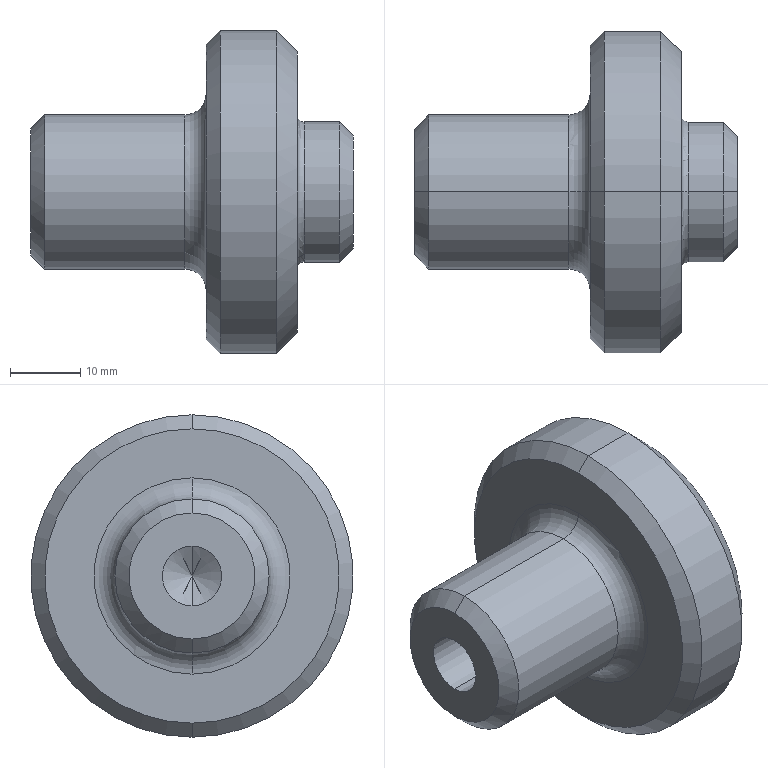Component | SolidWorks | THK-A1027LiftingMotorFlangeMountingAxis-1 | 1 solid | 26 faces | box 46 x 46 x 46 mm | volume 31160 mm3 | cone 10 | cylinder 8 | torus 4 | plane 4 | commonest cylinder face diameters 8.5 x2 22 x2 46 x2 20 x2 | material 45
build123d program:
from build123d import *

# Parameters (mm, degrees)
SKETCH1_R              = 10
BOSS_EXTRUDE1_DEPTH    = 4
SKETCH2_R              = 23
BOSS_EXTRUDE2_DEPTH    = 13
SKETCH3_R              = 11
BOSS_EXTRUDE3_DEPTH    = 25
M10_TAPPED_HOLE1_D     = 8.5
M10_TAPPED_HOLE1_DEPTH = 25
M10_TAPPED_HOLE1_TIP   = 2.554
CHAMFER1_SIZE          = 2
FILLET1_R              = 3
FILLET2_R              = 1
CHAMFER2_SIZE          = 3


with BuildPart() as part:
    # Sketch1 → Boss-Extrude1 (new, symmetric)
    with BuildSketch(Plane(origin=(0, 0, 0), x_dir=(0, 0, -1), z_dir=(1, 0, 0))):
        Circle(SKETCH1_R)
    extrude(amount=BOSS_EXTRUDE1_DEPTH, both=True)

    # Sketch2 → Boss-Extrude2 (add)
    with BuildSketch(Plane.ZY.offset(4)):
        with Locations(Location((0, 0, 0), (0, 0, 180))):
            Circle(SKETCH2_R)
    extrude(amount=BOSS_EXTRUDE2_DEPTH)

    # Sketch3 → Boss-Extrude3 (add)
    with BuildSketch(Plane.ZY.offset(17)):
        Circle(SKETCH3_R)
    extrude(amount=BOSS_EXTRUDE3_DEPTH)

    # M10 Tapped Hole1
    with Locations(Plane.ZY.offset(42)):
        with Locations((0, 0)):
            Hole(M10_TAPPED_HOLE1_D / 2, depth=M10_TAPPED_HOLE1_DEPTH)
            with Locations((0, 0, -(M10_TAPPED_HOLE1_DEPTH + M10_TAPPED_HOLE1_TIP / 2))):  # 118° drill point
                Cone(0, M10_TAPPED_HOLE1_D / 2, M10_TAPPED_HOLE1_TIP, mode=Mode.SUBTRACT)

    # Chamfer1
    chamfer1_edges = [part.edges().sort_by_distance(p)[0] for p in [
        (-42, 0, -11),
        (4, 0, 10),
        (-17, 0, 23),
    ]]
    chamfer(chamfer1_edges, length=CHAMFER1_SIZE)

    # Fillet1
    fillet1_edges = [part.edges().sort_by_distance(p)[0] for p in [
        (-17, 0, -11),
    ]]
    fillet(fillet1_edges, radius=FILLET1_R)

    # Fillet2
    fillet2_edges = [part.edges().sort_by_distance(p)[0] for p in [
        (-4, 0, 10),
    ]]
    fillet(fillet2_edges, radius=FILLET2_R)

    # Chamfer2
    chamfer2_edges = [part.edges().sort_by_distance(p)[0] for p in [
        (-4, 0, 23),
    ]]
    chamfer(chamfer2_edges, length=CHAMFER2_SIZE)


solid = part.part

# Placed as in the assembly
solid = solid.moved(Location((-120, 543, -50), (0, 0, 0)))
STEP:
#1=COLOUR_RGB('',0.7922,0.8196,0.9333);
#2=FILL_AREA_STYLE_COLOUR('',#1);
#3=FILL_AREA_STYLE('',(#2));
#4=SURFACE_STYLE_FILL_AREA(#3);
#5=SURFACE_SIDE_STYLE('',(#4));
#6=SURFACE_STYLE_USAGE(.BOTH.,#5);
#7=PRESENTATION_STYLE_ASSIGNMENT((#6));
#8=CARTESIAN_POINT('',(-4.882,21.378,-2.756));
#9=VERTEX_POINT('',#8);
#10=CARTESIAN_POINT('',(-4.882,21.378,-1.181));
#11=VERTEX_POINT('',#10);
#12=CARTESIAN_POINT('',(-4.882,21.378,-1.969));
#13=DIRECTION('',(1.,0.,0.));
#14=DIRECTION('',(0.,0.,1.));
#15=AXIS2_PLACEMENT_3D('',#12,#13,#14);
#16=CIRCLE('',#15,0.7874);
#17=EDGE_CURVE('',#9,#11,#16,.T.);
#18=ORIENTED_EDGE('',*,*,#17,.F.);
#19=CARTESIAN_POINT('',(-5.,21.378,-2.874));
#20=VERTEX_POINT('',#19);
#21=CARTESIAN_POINT('',(-5.,21.378,-2.874));
#22=DIRECTION('',(-0.7071,0.,-0.7071));
#23=VECTOR('',#22,39.37);
#24=LINE('',#21,#23);
#25=EDGE_CURVE('',#9,#20,#24,.T.);
#26=ORIENTED_EDGE('',*,*,#25,.T.);
#27=CARTESIAN_POINT('',(-5.,21.378,-1.063));
#28=VERTEX_POINT('',#27);
#29=CARTESIAN_POINT('',(-5.,21.378,-1.969));
#30=DIRECTION('',(-1.,0.,-0.));
#31=DIRECTION('',(0.,0.,1.));
#32=AXIS2_PLACEMENT_3D('',#29,#30,#31);
#33=CIRCLE('',#32,0.9055);
#34=EDGE_CURVE('',#28,#20,#33,.T.);
#35=ORIENTED_EDGE('',*,*,#34,.F.);
#36=CARTESIAN_POINT('',(-5.,21.378,-1.063));
#37=DIRECTION('',(-0.7071,0.,0.7071));
#38=VECTOR('',#37,39.37);
#39=LINE('',#36,#38);
#40=EDGE_CURVE('',#11,#28,#39,.T.);
#41=ORIENTED_EDGE('',*,*,#40,.F.);
#42=EDGE_LOOP('',(#18,#26,#35,#41));
#43=FACE_OUTER_BOUND('',#42,.T.);
#44=CARTESIAN_POINT('',(-5.,21.378,-1.969));
#45=DIRECTION('',(-1.,0.,-0.));
#46=DIRECTION('',(0.,0.,1.));
#47=AXIS2_PLACEMENT_3D('',#44,#45,#46);
#48=CONICAL_SURFACE('',#47,0.9055,0.7854);
#49=ADVANCED_FACE('',(#43),#48,.T.);
#50=CARTESIAN_POINT('',(-4.882,21.378,-2.402));
#51=VERTEX_POINT('',#50);
#52=CARTESIAN_POINT('',(-4.882,21.378,-1.535));
#53=VERTEX_POINT('',#52);
#54=CARTESIAN_POINT('',(-4.882,21.378,-1.969));
#55=DIRECTION('',(-1.,0.,-0.));
#56=DIRECTION('',(0.,0.,1.));
#57=AXIS2_PLACEMENT_3D('',#54,#55,#56);
#58=CIRCLE('',#57,0.4331);
#59=EDGE_CURVE('',#51,#53,#58,.T.);
#60=ORIENTED_EDGE('',*,*,#59,.F.);
#61=CARTESIAN_POINT('',(-4.843,21.378,-2.362));
#62=VERTEX_POINT('',#61);
#63=CARTESIAN_POINT('',(-4.843,21.378,-2.402));
#64=DIRECTION('',(-0.,1.,0.));
#65=DIRECTION('',(0.,0.,1.));
#66=AXIS2_PLACEMENT_3D('',#63,#64,#65);
#67=CIRCLE('',#66,0.03937);
#68=EDGE_CURVE('',#51,#62,#67,.T.);
#69=ORIENTED_EDGE('',*,*,#68,.T.);
#70=CARTESIAN_POINT('',(-4.843,21.378,-1.575));
#71=VERTEX_POINT('',#70);
#72=CARTESIAN_POINT('',(-4.843,21.378,-1.969));
#73=DIRECTION('',(1.,0.,0.));
#74=DIRECTION('',(0.,0.,1.));
#75=AXIS2_PLACEMENT_3D('',#72,#73,#74);
#76=CIRCLE('',#75,0.3937);
#77=EDGE_CURVE('',#71,#62,#76,.T.);
#78=ORIENTED_EDGE('',*,*,#77,.F.);
#79=CARTESIAN_POINT('',(-4.843,21.378,-1.535));
#80=DIRECTION('',(0.,-1.,0.));
#81=DIRECTION('',(0.,0.,-1.));
#82=AXIS2_PLACEMENT_3D('',#79,#80,#81);
#83=CIRCLE('',#82,0.03937);
#84=EDGE_CURVE('',#53,#71,#83,.T.);
#85=ORIENTED_EDGE('',*,*,#84,.F.);
#86=EDGE_LOOP('',(#60,#69,#78,#85));
#87=FACE_OUTER_BOUND('',#86,.T.);
#88=CARTESIAN_POINT('',(-4.843,21.378,-1.969));
#89=DIRECTION('',(-1.,0.,-0.));
#90=DIRECTION('',(-0.,0.,1.));
#91=AXIS2_PLACEMENT_3D('',#88,#89,#90);
#92=TOROIDAL_SURFACE('',#91,0.4331,0.03937);
#93=ADVANCED_FACE('',(#87),#92,.F.);
#94=CARTESIAN_POINT('',(-5.512,21.378,-2.402));
#95=VERTEX_POINT('',#94);
#96=CARTESIAN_POINT('',(-5.512,21.378,-1.535));
#97=VERTEX_POINT('',#96);
#98=CARTESIAN_POINT('',(-5.512,21.378,-1.969));
#99=DIRECTION('',(-1.,0.,-0.));
#100=DIRECTION('',(0.,0.,1.));
#101=AXIS2_PLACEMENT_3D('',#98,#99,#100);
#102=CIRCLE('',#101,0.4331);
#103=EDGE_CURVE('',#95,#97,#102,.T.);
#104=ORIENTED_EDGE('',*,*,#103,.F.);
#105=CARTESIAN_POINT('',(-5.394,21.378,-2.52));
#106=VERTEX_POINT('',#105);
#107=CARTESIAN_POINT('',(-5.512,21.378,-2.52));
#108=DIRECTION('',(-0.,1.,0.));
#109=DIRECTION('',(0.,0.,1.));
#110=AXIS2_PLACEMENT_3D('',#107,#108,#109);
#111=CIRCLE('',#110,0.1181);
#112=EDGE_CURVE('',#95,#106,#111,.T.);
#113=ORIENTED_EDGE('',*,*,#112,.T.);
#114=CARTESIAN_POINT('',(-5.394,21.378,-1.417));
#115=VERTEX_POINT('',#114);
#116=CARTESIAN_POINT('',(-5.394,21.378,-1.969));
#117=DIRECTION('',(1.,0.,0.));
#118=DIRECTION('',(0.,0.,1.));
#119=AXIS2_PLACEMENT_3D('',#116,#117,#118);
#120=CIRCLE('',#119,0.5512);
#121=EDGE_CURVE('',#115,#106,#120,.T.);
#122=ORIENTED_EDGE('',*,*,#121,.F.);
#123=CARTESIAN_POINT('',(-5.512,21.378,-1.417));
#124=DIRECTION('',(0.,-1.,0.));
#125=DIRECTION('',(0.,0.,-1.));
#126=AXIS2_PLACEMENT_3D('',#123,#124,#125);
#127=CIRCLE('',#126,0.1181);
#128=EDGE_CURVE('',#97,#115,#127,.T.);
#129=ORIENTED_EDGE('',*,*,#128,.F.);
#130=EDGE_LOOP('',(#104,#113,#122,#129));
#131=FACE_OUTER_BOUND('',#130,.T.);
#132=CARTESIAN_POINT('',(-5.512,21.378,-1.969));
#133=DIRECTION('',(-1.,0.,-0.));
#134=DIRECTION('',(-0.,0.,1.));
#135=AXIS2_PLACEMENT_3D('',#132,#133,#134);
#136=TOROIDAL_SURFACE('',#135,0.5512,0.1181);
#137=ADVANCED_FACE('',(#131),#136,.F.);
#138=CARTESIAN_POINT('',(-4.567,21.378,-2.283));
#139=VERTEX_POINT('',#138);
#140=CARTESIAN_POINT('',(-4.567,21.378,-1.654));
#141=VERTEX_POINT('',#140);
#142=CARTESIAN_POINT('',(-4.567,21.378,-1.969));
#143=DIRECTION('',(1.,0.,0.));
#144=DIRECTION('',(0.,0.,-1.));
#145=AXIS2_PLACEMENT_3D('',#142,#143,#144);
#146=CIRCLE('',#145,0.315);
#147=EDGE_CURVE('',#139,#141,#146,.T.);
#148=ORIENTED_EDGE('',*,*,#147,.F.);
#149=CARTESIAN_POINT('',(-4.646,21.378,-2.362));
#150=VERTEX_POINT('',#149);
#151=CARTESIAN_POINT('',(-4.567,21.378,-2.283));
#152=DIRECTION('',(-0.7071,0.,-0.7071));
#153=VECTOR('',#152,39.37);
#154=LINE('',#151,#153);
#155=EDGE_CURVE('',#139,#150,#154,.T.);
#156=ORIENTED_EDGE('',*,*,#155,.T.);
#157=CARTESIAN_POINT('',(-4.646,21.378,-1.575));
#158=VERTEX_POINT('',#157);
#159=CARTESIAN_POINT('',(-4.646,21.378,-1.969));
#160=DIRECTION('',(-1.,0.,0.));
#161=DIRECTION('',(0.,0.,-1.));
#162=AXIS2_PLACEMENT_3D('',#159,#160,#161);
#163=CIRCLE('',#162,0.3937);
#164=EDGE_CURVE('',#158,#150,#163,.T.);
#165=ORIENTED_EDGE('',*,*,#164,.F.);
#166=CARTESIAN_POINT('',(-4.567,21.378,-1.654));
#167=DIRECTION('',(-0.7071,0.,0.7071));
#168=VECTOR('',#167,39.37);
#169=LINE('',#166,#168);
#170=EDGE_CURVE('',#141,#158,#169,.T.);
#171=ORIENTED_EDGE('',*,*,#170,.F.);
#172=EDGE_LOOP('',(#148,#156,#165,#171));
#173=FACE_OUTER_BOUND('',#172,.T.);
#174=CARTESIAN_POINT('',(-4.567,21.378,-1.969));
#175=DIRECTION('',(-1.,0.,0.));
#176=DIRECTION('',(0.,0.,1.));
#177=AXIS2_PLACEMENT_3D('',#174,#175,#176);
#178=CONICAL_SURFACE('',#177,0.315,0.7854);
#179=ADVANCED_FACE('',(#173),#178,.T.);
#180=CARTESIAN_POINT('',(-5.394,21.378,-1.142));
#181=VERTEX_POINT('',#180);
#182=CARTESIAN_POINT('',(-5.394,21.378,-2.795));
#183=VERTEX_POINT('',#182);
#184=CARTESIAN_POINT('',(-5.394,21.378,-1.969));
#185=DIRECTION('',(-1.,0.,-0.));
#186=DIRECTION('',(0.,0.,1.));
#187=AXIS2_PLACEMENT_3D('',#184,#185,#186);
#188=CIRCLE('',#187,0.8268);
#189=EDGE_CURVE('',#181,#183,#188,.T.);
#190=ORIENTED_EDGE('',*,*,#189,.F.);
#191=CARTESIAN_POINT('',(-5.315,21.378,-1.063));
#192=VERTEX_POINT('',#191);
#193=CARTESIAN_POINT('',(-5.394,21.378,-1.142));
#194=DIRECTION('',(0.7071,0.,0.7071));
#195=VECTOR('',#194,39.37);
#196=LINE('',#193,#195);
#197=EDGE_CURVE('',#181,#192,#196,.T.);
#198=ORIENTED_EDGE('',*,*,#197,.T.);
#199=CARTESIAN_POINT('',(-5.315,21.378,-2.874));
#200=VERTEX_POINT('',#199);
#201=CARTESIAN_POINT('',(-5.315,21.378,-1.969));
#202=DIRECTION('',(1.,0.,0.));
#203=DIRECTION('',(0.,0.,1.));
#204=AXIS2_PLACEMENT_3D('',#201,#202,#203);
#205=CIRCLE('',#204,0.9055);
#206=EDGE_CURVE('',#200,#192,#205,.T.);
#207=ORIENTED_EDGE('',*,*,#206,.F.);
#208=CARTESIAN_POINT('',(-5.394,21.378,-2.795));
#209=DIRECTION('',(0.7071,0.,-0.7071));
#210=VECTOR('',#209,39.37);
#211=LINE('',#208,#210);
#212=EDGE_CURVE('',#183,#200,#211,.T.);
#213=ORIENTED_EDGE('',*,*,#212,.F.);
#214=EDGE_LOOP('',(#190,#198,#207,#213));
#215=FACE_OUTER_BOUND('',#214,.T.);
#216=CARTESIAN_POINT('',(-5.394,21.378,-1.969));
#217=DIRECTION('',(1.,0.,0.));
#218=DIRECTION('',(0.,0.,-1.));
#219=AXIS2_PLACEMENT_3D('',#216,#217,#218);
#220=CONICAL_SURFACE('',#219,0.8268,0.7854);
#221=ADVANCED_FACE('',(#215),#220,.T.);
#222=CARTESIAN_POINT('',(-6.378,21.378,-1.614));
#223=VERTEX_POINT('',#222);
#224=CARTESIAN_POINT('',(-6.378,21.378,-2.323));
#225=VERTEX_POINT('',#224);
#226=CARTESIAN_POINT('',(-6.378,21.378,-1.969));
#227=DIRECTION('',(-1.,0.,-0.));
#228=DIRECTION('',(0.,0.,1.));
#229=AXIS2_PLACEMENT_3D('',#226,#227,#228);
#230=CIRCLE('',#229,0.3543);
#231=EDGE_CURVE('',#223,#225,#230,.T.);
#232=ORIENTED_EDGE('',*,*,#231,.F.);
#233=CARTESIAN_POINT('',(-6.299,21.378,-1.535));
#234=VERTEX_POINT('',#233);
#235=CARTESIAN_POINT('',(-6.378,21.378,-1.614));
#236=DIRECTION('',(0.7071,0.,0.7071));
#237=VECTOR('',#236,39.37);
#238=LINE('',#235,#237);
#239=EDGE_CURVE('',#223,#234,#238,.T.);
#240=ORIENTED_EDGE('',*,*,#239,.T.);
#241=CARTESIAN_POINT('',(-6.299,21.378,-2.402));
#242=VERTEX_POINT('',#241);
#243=CARTESIAN_POINT('',(-6.299,21.378,-1.969));
#244=DIRECTION('',(1.,0.,0.));
#245=DIRECTION('',(0.,0.,1.));
#246=AXIS2_PLACEMENT_3D('',#243,#244,#245);
#247=CIRCLE('',#246,0.4331);
#248=EDGE_CURVE('',#242,#234,#247,.T.);
#249=ORIENTED_EDGE('',*,*,#248,.F.);
#250=CARTESIAN_POINT('',(-6.378,21.378,-2.323));
#251=DIRECTION('',(0.7071,0.,-0.7071));
#252=VECTOR('',#251,39.37);
#253=LINE('',#250,#252);
#254=EDGE_CURVE('',#225,#242,#253,.T.);
#255=ORIENTED_EDGE('',*,*,#254,.F.);
#256=EDGE_LOOP('',(#232,#240,#249,#255));
#257=FACE_OUTER_BOUND('',#256,.T.);
#258=CARTESIAN_POINT('',(-6.378,21.378,-1.969));
#259=DIRECTION('',(1.,0.,0.));
#260=DIRECTION('',(0.,0.,-1.));
#261=AXIS2_PLACEMENT_3D('',#258,#259,#260);
#262=CONICAL_SURFACE('',#261,0.3543,0.7854);
#263=ADVANCED_FACE('',(#257),#262,.T.);
#264=CARTESIAN_POINT('',(-5.394,21.378,-2.136));
#265=VERTEX_POINT('',#264);
#266=CARTESIAN_POINT('',(-5.394,21.378,-1.801));
#267=VERTEX_POINT('',#266);
#268=CARTESIAN_POINT('',(-5.394,21.378,-1.969));
#269=DIRECTION('',(-1.,0.,-0.));
#270=DIRECTION('',(0.,0.,1.));
#271=AXIS2_PLACEMENT_3D('',#268,#269,#270);
#272=CIRCLE('',#271,0.1673);
#273=EDGE_CURVE('',#265,#267,#272,.T.);
#274=ORIENTED_EDGE('',*,*,#273,.F.);
#275=CARTESIAN_POINT('',(-6.378,21.378,-2.136));
#276=VERTEX_POINT('',#275);
#277=CARTESIAN_POINT('',(-6.378,21.378,-2.136));
#278=DIRECTION('',(-1.,0.,-0.));
#279=VECTOR('',#278,39.37);
#280=LINE('',#277,#279);
#281=EDGE_CURVE('',#265,#276,#280,.T.);
#282=ORIENTED_EDGE('',*,*,#281,.T.);
#283=CARTESIAN_POINT('',(-6.378,21.378,-1.801));
#284=VERTEX_POINT('',#283);
#285=CARTESIAN_POINT('',(-6.378,21.378,-1.969));
#286=DIRECTION('',(-1.,0.,-0.));
#287=DIRECTION('',(0.,0.,1.));
#288=AXIS2_PLACEMENT_3D('',#285,#286,#287);
#289=CIRCLE('',#288,0.1673);
#290=EDGE_CURVE('',#276,#284,#289,.T.);
#291=ORIENTED_EDGE('',*,*,#290,.T.);
#292=CARTESIAN_POINT('',(-6.378,21.378,-1.801));
#293=DIRECTION('',(-1.,0.,-0.));
#294=VECTOR('',#293,39.37);
#295=LINE('',#292,#294);
#296=EDGE_CURVE('',#267,#284,#295,.T.);
#297=ORIENTED_EDGE('',*,*,#296,.F.);
#298=EDGE_LOOP('',(#274,#282,#291,#297));
#299=FACE_OUTER_BOUND('',#298,.T.);
#300=CARTESIAN_POINT('',(-6.378,21.378,-1.969));
#301=DIRECTION('',(-1.,0.,-0.));
#302=DIRECTION('',(0.,0.,1.));
#303=AXIS2_PLACEMENT_3D('',#300,#301,#302);
#304=CYLINDRICAL_SURFACE('',#303,0.1673);
#305=ADVANCED_FACE('',(#299),#304,.F.);
#306=CARTESIAN_POINT('',(-5.293,21.378,-1.969));
#307=VERTEX_POINT('',#306);
#308=CARTESIAN_POINT('',(-5.394,21.378,-1.801));
#309=DIRECTION('',(-0.515,0.,0.8572));
#310=VECTOR('',#309,39.37);
#311=LINE('',#308,#310);
#312=EDGE_CURVE('',#307,#267,#311,.T.);
#313=ORIENTED_EDGE('',*,*,#312,.F.);
#314=CARTESIAN_POINT('',(-5.394,21.378,-2.136));
#315=DIRECTION('',(-0.515,0.,-0.8572));
#316=VECTOR('',#315,39.37);
#317=LINE('',#314,#316);
#318=EDGE_CURVE('',#307,#265,#317,.T.);
#319=ORIENTED_EDGE('',*,*,#318,.T.);
#320=ORIENTED_EDGE('',*,*,#273,.T.);
#321=EDGE_LOOP('',(#313,#319,#320));
#322=FACE_OUTER_BOUND('',#321,.T.);
#323=CARTESIAN_POINT('',(-5.394,21.378,-1.969));
#324=DIRECTION('',(-1.,0.,-0.));
#325=DIRECTION('',(0.,0.,1.));
#326=AXIS2_PLACEMENT_3D('',#323,#324,#325);
#327=CONICAL_SURFACE('',#326,0.1673,1.03);
#328=ADVANCED_FACE('',(#322),#327,.F.);
#329=ORIENTED_EDGE('',*,*,#248,.T.);
#330=CARTESIAN_POINT('',(-6.378,21.378,-1.535));
#331=DIRECTION('',(1.,0.,0.));
#332=VECTOR('',#331,39.37);
#333=LINE('',#330,#332);
#334=EDGE_CURVE('',#234,#97,#333,.T.);
#335=ORIENTED_EDGE('',*,*,#334,.T.);
#336=CARTESIAN_POINT('',(-5.512,21.378,-1.969));
#337=DIRECTION('',(-1.,0.,-0.));
#338=DIRECTION('',(0.,0.,1.));
#339=AXIS2_PLACEMENT_3D('',#336,#337,#338);
#340=CIRCLE('',#339,0.4331);
#341=EDGE_CURVE('',#97,#95,#340,.T.);
#342=ORIENTED_EDGE('',*,*,#341,.T.);
#343=CARTESIAN_POINT('',(-6.378,21.378,-2.402));
#344=DIRECTION('',(1.,0.,0.));
#345=VECTOR('',#344,39.37);
#346=LINE('',#343,#345);
#347=EDGE_CURVE('',#242,#95,#346,.T.);
#348=ORIENTED_EDGE('',*,*,#347,.F.);
#349=EDGE_LOOP('',(#329,#335,#342,#348));
#350=FACE_OUTER_BOUND('',#349,.T.);
#351=CARTESIAN_POINT('',(-6.378,21.378,-1.969));
#352=DIRECTION('',(1.,0.,0.));
#353=DIRECTION('',(0.,0.,-1.));
#354=AXIS2_PLACEMENT_3D('',#351,#352,#353);
#355=CYLINDRICAL_SURFACE('',#354,0.4331);
#356=ADVANCED_FACE('',(#350),#355,.T.);
#357=ORIENTED_EDGE('',*,*,#206,.T.);
#358=CARTESIAN_POINT('',(-5.394,21.378,-1.063));
#359=DIRECTION('',(1.,0.,0.));
#360=VECTOR('',#359,39.37);
#361=LINE('',#358,#360);
#362=EDGE_CURVE('',#192,#28,#361,.T.);
#363=ORIENTED_EDGE('',*,*,#362,.T.);
#364=ORIENTED_EDGE('',*,*,#34,.T.);
#365=CARTESIAN_POINT('',(-5.394,21.378,-2.874));
#366=DIRECTION('',(1.,0.,0.));
#367=VECTOR('',#366,39.37);
#368=LINE('',#365,#367);
#369=EDGE_CURVE('',#200,#20,#368,.T.);
#370=ORIENTED_EDGE('',*,*,#369,.F.);
#371=EDGE_LOOP('',(#357,#363,#364,#370));
#372=FACE_OUTER_BOUND('',#371,.T.);
#373=CARTESIAN_POINT('',(-5.394,21.378,-1.969));
#374=DIRECTION('',(1.,0.,0.));
#375=DIRECTION('',(0.,0.,-1.));
#376=AXIS2_PLACEMENT_3D('',#373,#374,#375);
#377=CYLINDRICAL_SURFACE('',#376,0.9055);
#378=ADVANCED_FACE('',(#372),#377,.T.);
#379=ORIENTED_EDGE('',*,*,#164,.T.);
#380=CARTESIAN_POINT('',(-4.567,21.378,-2.362));
#381=DIRECTION('',(-1.,0.,0.));
#382=VECTOR('',#381,39.37);
#383=LINE('',#380,#382);
#384=EDGE_CURVE('',#150,#62,#383,.T.);
#385=ORIENTED_EDGE('',*,*,#384,.T.);
#386=CARTESIAN_POINT('',(-4.843,21.378,-1.969));
#387=DIRECTION('',(1.,0.,0.));
#388=DIRECTION('',(0.,0.,1.));
#389=AXIS2_PLACEMENT_3D('',#386,#387,#388);
#390=CIRCLE('',#389,0.3937);
#391=EDGE_CURVE('',#62,#71,#390,.T.);
#392=ORIENTED_EDGE('',*,*,#391,.T.);
#393=CARTESIAN_POINT('',(-4.567,21.378,-1.575));
#394=DIRECTION('',(-1.,0.,0.));
#395=VECTOR('',#394,39.37);
#396=LINE('',#393,#395);
#397=EDGE_CURVE('',#158,#71,#396,.T.);
#398=ORIENTED_EDGE('',*,*,#397,.F.);
#399=EDGE_LOOP('',(#379,#385,#392,#398));
#400=FACE_OUTER_BOUND('',#399,.T.);
#401=CARTESIAN_POINT('',(-4.567,21.378,-1.969));
#402=DIRECTION('',(-1.,0.,0.));
#403=DIRECTION('',(0.,0.,1.));
#404=AXIS2_PLACEMENT_3D('',#401,#402,#403);
#405=CYLINDRICAL_SURFACE('',#404,0.3937);
#406=ADVANCED_FACE('',(#400),#405,.T.);
#407=ORIENTED_EDGE('',*,*,#121,.T.);
#408=CARTESIAN_POINT('',(-5.394,21.378,-1.969));
#409=DIRECTION('',(1.,0.,0.));
#410=DIRECTION('',(0.,0.,1.));
#411=AXIS2_PLACEMENT_3D('',#408,#409,#410);
#412=CIRCLE('',#411,0.5512);
#413=EDGE_CURVE('',#106,#115,#412,.T.);
#414=ORIENTED_EDGE('',*,*,#413,.T.);
#415=EDGE_LOOP('',(#407,#414));
#416=FACE_BOUND('',#415,.T.);
#417=CARTESIAN_POINT('',(-5.394,21.378,-1.969));
#418=DIRECTION('',(-1.,0.,-0.));
#419=DIRECTION('',(0.,0.,1.));
#420=AXIS2_PLACEMENT_3D('',#417,#418,#419);
#421=CIRCLE('',#420,0.8268);
#422=EDGE_CURVE('',#183,#181,#421,.T.);
#423=ORIENTED_EDGE('',*,*,#422,.T.);
#424=ORIENTED_EDGE('',*,*,#189,.T.);
#425=EDGE_LOOP('',(#423,#424));
#426=FACE_OUTER_BOUND('',#425,.T.);
#427=CARTESIAN_POINT('',(-5.394,21.378,-1.969));
#428=DIRECTION('',(-1.,0.,-0.));
#429=DIRECTION('',(-0.,0.,1.));
#430=AXIS2_PLACEMENT_3D('',#427,#428,#429);
#431=PLANE('',#430);
#432=ADVANCED_FACE('',(#416,#426),#431,.T.);
#433=ORIENTED_EDGE('',*,*,#384,.F.);
#434=CARTESIAN_POINT('',(-4.646,21.378,-1.969));
#435=DIRECTION('',(-1.,0.,0.));
#436=DIRECTION('',(0.,0.,-1.));
#437=AXIS2_PLACEMENT_3D('',#434,#435,#436);
#438=CIRCLE('',#437,0.3937);
#439=EDGE_CURVE('',#150,#158,#438,.T.);
#440=ORIENTED_EDGE('',*,*,#439,.T.);
#441=ORIENTED_EDGE('',*,*,#397,.T.);
#442=ORIENTED_EDGE('',*,*,#77,.T.);
#443=EDGE_LOOP('',(#433,#440,#441,#442));
#444=FACE_OUTER_BOUND('',#443,.T.);
#445=CARTESIAN_POINT('',(-4.567,21.378,-1.969));
#446=DIRECTION('',(-1.,0.,0.));
#447=DIRECTION('',(0.,0.,1.));
#448=AXIS2_PLACEMENT_3D('',#445,#446,#447);
#449=CYLINDRICAL_SURFACE('',#448,0.3937);
#450=ADVANCED_FACE('',(#444),#449,.T.);
#451=CARTESIAN_POINT('',(-4.567,21.378,-1.969));
#452=DIRECTION('',(1.,0.,0.));
#453=DIRECTION('',(0.,0.,-1.));
#454=AXIS2_PLACEMENT_3D('',#451,#452,#453);
#455=CIRCLE('',#454,0.315);
#456=EDGE_CURVE('',#141,#139,#455,.T.);
#457=ORIENTED_EDGE('',*,*,#456,.T.);
#458=ORIENTED_EDGE('',*,*,#147,.T.);
#459=EDGE_LOOP('',(#457,#458));
#460=FACE_OUTER_BOUND('',#459,.T.);
#461=CARTESIAN_POINT('',(-4.567,21.378,-1.969));
#462=DIRECTION('',(1.,0.,0.));
#463=DIRECTION('',(0.,0.,-1.));
#464=AXIS2_PLACEMENT_3D('',#461,#462,#463);
#465=PLANE('',#464);
#466=ADVANCED_FACE('',(#460),#465,.T.);
#467=CARTESIAN_POINT('',(-4.882,21.378,-1.969));
#468=DIRECTION('',(1.,0.,0.));
#469=DIRECTION('',(0.,0.,1.));
#470=AXIS2_PLACEMENT_3D('',#467,#468,#469);
#471=CIRCLE('',#470,0.7874);
#472=EDGE_CURVE('',#11,#9,#471,.T.);
#473=ORIENTED_EDGE('',*,*,#472,.T.);
#474=ORIENTED_EDGE('',*,*,#17,.T.);
#475=EDGE_LOOP('',(#473,#474));
#476=FACE_OUTER_BOUND('',#475,.T.);
#477=CARTESIAN_POINT('',(-4.882,21.378,-1.969));
#478=DIRECTION('',(-1.,0.,-0.));
#479=DIRECTION('',(0.,0.,1.));
#480=AXIS2_PLACEMENT_3D('',#477,#478,#479);
#481=CIRCLE('',#480,0.4331);
#482=EDGE_CURVE('',#53,#51,#481,.T.);
#483=ORIENTED_EDGE('',*,*,#482,.T.);
#484=ORIENTED_EDGE('',*,*,#59,.T.);
#485=EDGE_LOOP('',(#483,#484));
#486=FACE_BOUND('',#485,.T.);
#487=CARTESIAN_POINT('',(-4.882,21.378,-1.969));
#488=DIRECTION('',(-1.,0.,-0.));
#489=DIRECTION('',(-0.,0.,1.));
#490=AXIS2_PLACEMENT_3D('',#487,#488,#489);
#491=PLANE('',#490);
#492=ADVANCED_FACE('',(#476,#486),#491,.F.);
#493=ORIENTED_EDGE('',*,*,#362,.F.);
#494=CARTESIAN_POINT('',(-5.315,21.378,-1.969));
#495=DIRECTION('',(1.,0.,0.));
#496=DIRECTION('',(0.,0.,1.));
#497=AXIS2_PLACEMENT_3D('',#494,#495,#496);
#498=CIRCLE('',#497,0.9055);
#499=EDGE_CURVE('',#192,#200,#498,.T.);
#500=ORIENTED_EDGE('',*,*,#499,.T.);
#501=ORIENTED_EDGE('',*,*,#369,.T.);
#502=CARTESIAN_POINT('',(-5.,21.378,-1.969));
#503=DIRECTION('',(-1.,0.,-0.));
#504=DIRECTION('',(0.,0.,1.));
#505=AXIS2_PLACEMENT_3D('',#502,#503,#504);
#506=CIRCLE('',#505,0.9055);
#507=EDGE_CURVE('',#20,#28,#506,.T.);
#508=ORIENTED_EDGE('',*,*,#507,.T.);
#509=EDGE_LOOP('',(#493,#500,#501,#508));
#510=FACE_OUTER_BOUND('',#509,.T.);
#511=CARTESIAN_POINT('',(-5.394,21.378,-1.969));
#512=DIRECTION('',(1.,0.,0.));
#513=DIRECTION('',(0.,0.,-1.));
#514=AXIS2_PLACEMENT_3D('',#511,#512,#513);
#515=CYLINDRICAL_SURFACE('',#514,0.9055);
#516=ADVANCED_FACE('',(#510),#515,.T.);
#517=ORIENTED_EDGE('',*,*,#334,.F.);
#518=CARTESIAN_POINT('',(-6.299,21.378,-1.969));
#519=DIRECTION('',(1.,0.,0.));
#520=DIRECTION('',(0.,0.,1.));
#521=AXIS2_PLACEMENT_3D('',#518,#519,#520);
#522=CIRCLE('',#521,0.4331);
#523=EDGE_CURVE('',#234,#242,#522,.T.);
#524=ORIENTED_EDGE('',*,*,#523,.T.);
#525=ORIENTED_EDGE('',*,*,#347,.T.);
#526=ORIENTED_EDGE('',*,*,#103,.T.);
#527=EDGE_LOOP('',(#517,#524,#525,#526));
#528=FACE_OUTER_BOUND('',#527,.T.);
#529=CARTESIAN_POINT('',(-6.378,21.378,-1.969));
#530=DIRECTION('',(1.,0.,0.));
#531=DIRECTION('',(0.,0.,-1.));
#532=AXIS2_PLACEMENT_3D('',#529,#530,#531);
#533=CYLINDRICAL_SURFACE('',#532,0.4331);
#534=ADVANCED_FACE('',(#528),#533,.T.);
#535=CARTESIAN_POINT('',(-6.378,21.378,-1.969));
#536=DIRECTION('',(-1.,0.,-0.));
#537=DIRECTION('',(0.,0.,1.));
#538=AXIS2_PLACEMENT_3D('',#535,#536,#537);
#539=CIRCLE('',#538,0.3543);
#540=EDGE_CURVE('',#225,#223,#539,.T.);
#541=ORIENTED_EDGE('',*,*,#540,.T.);
#542=ORIENTED_EDGE('',*,*,#231,.T.);
#543=EDGE_LOOP('',(#541,#542));
#544=FACE_OUTER_BOUND('',#543,.T.);
#545=CARTESIAN_POINT('',(-6.378,21.378,-1.969));
#546=DIRECTION('',(-1.,0.,-0.));
#547=DIRECTION('',(0.,0.,1.));
#548=AXIS2_PLACEMENT_3D('',#545,#546,#547);
#549=CIRCLE('',#548,0.1673);
#550=EDGE_CURVE('',#284,#276,#549,.T.);
#551=ORIENTED_EDGE('',*,*,#550,.F.);
#552=ORIENTED_EDGE('',*,*,#290,.F.);
#553=EDGE_LOOP('',(#551,#552));
#554=FACE_BOUND('',#553,.T.);
#555=CARTESIAN_POINT('',(-6.378,21.378,-1.969));
#556=DIRECTION('',(-1.,0.,-0.));
#557=DIRECTION('',(-0.,0.,1.));
#558=AXIS2_PLACEMENT_3D('',#555,#556,#557);
#559=PLANE('',#558);
#560=ADVANCED_FACE('',(#544,#554),#559,.T.);
#561=ORIENTED_EDGE('',*,*,#318,.F.);
#562=ORIENTED_EDGE('',*,*,#312,.T.);
#563=CARTESIAN_POINT('',(-5.394,21.378,-1.969));
#564=DIRECTION('',(-1.,0.,-0.));
#565=DIRECTION('',(0.,0.,1.));
#566=AXIS2_PLACEMENT_3D('',#563,#564,#565);
#567=CIRCLE('',#566,0.1673);
#568=EDGE_CURVE('',#267,#265,#567,.T.);
#569=ORIENTED_EDGE('',*,*,#568,.T.);
#570=EDGE_LOOP('',(#561,#562,#569));
#571=FACE_OUTER_BOUND('',#570,.T.);
#572=CARTESIAN_POINT('',(-5.394,21.378,-1.969));
#573=DIRECTION('',(-1.,0.,-0.));
#574=DIRECTION('',(0.,0.,1.));
#575=AXIS2_PLACEMENT_3D('',#572,#573,#574);
#576=CONICAL_SURFACE('',#575,0.1673,1.03);
#577=ADVANCED_FACE('',(#571),#576,.F.);
#578=ORIENTED_EDGE('',*,*,#281,.F.);
#579=ORIENTED_EDGE('',*,*,#568,.F.);
#580=ORIENTED_EDGE('',*,*,#296,.T.);
#581=ORIENTED_EDGE('',*,*,#550,.T.);
#582=EDGE_LOOP('',(#578,#579,#580,#581));
#583=FACE_OUTER_BOUND('',#582,.T.);
#584=CARTESIAN_POINT('',(-6.378,21.378,-1.969));
#585=DIRECTION('',(-1.,0.,-0.));
#586=DIRECTION('',(0.,0.,1.));
#587=AXIS2_PLACEMENT_3D('',#584,#585,#586);
#588=CYLINDRICAL_SURFACE('',#587,0.1673);
#589=ADVANCED_FACE('',(#583),#588,.F.);
#590=ORIENTED_EDGE('',*,*,#239,.F.);
#591=ORIENTED_EDGE('',*,*,#540,.F.);
#592=ORIENTED_EDGE('',*,*,#254,.T.);
#593=ORIENTED_EDGE('',*,*,#523,.F.);
#594=EDGE_LOOP('',(#590,#591,#592,#593));
#595=FACE_OUTER_BOUND('',#594,.T.);
#596=CARTESIAN_POINT('',(-6.378,21.378,-1.969));
#597=DIRECTION('',(1.,0.,0.));
#598=DIRECTION('',(0.,0.,-1.));
#599=AXIS2_PLACEMENT_3D('',#596,#597,#598);
#600=CONICAL_SURFACE('',#599,0.3543,0.7854);
#601=ADVANCED_FACE('',(#595),#600,.T.);
#602=ORIENTED_EDGE('',*,*,#197,.F.);
#603=ORIENTED_EDGE('',*,*,#422,.F.);
#604=ORIENTED_EDGE('',*,*,#212,.T.);
#605=ORIENTED_EDGE('',*,*,#499,.F.);
#606=EDGE_LOOP('',(#602,#603,#604,#605));
#607=FACE_OUTER_BOUND('',#606,.T.);
#608=CARTESIAN_POINT('',(-5.394,21.378,-1.969));
#609=DIRECTION('',(1.,0.,0.));
#610=DIRECTION('',(0.,0.,-1.));
#611=AXIS2_PLACEMENT_3D('',#608,#609,#610);
#612=CONICAL_SURFACE('',#611,0.8268,0.7854);
#613=ADVANCED_FACE('',(#607),#612,.T.);
#614=ORIENTED_EDGE('',*,*,#155,.F.);
#615=ORIENTED_EDGE('',*,*,#456,.F.);
#616=ORIENTED_EDGE('',*,*,#170,.T.);
#617=ORIENTED_EDGE('',*,*,#439,.F.);
#618=EDGE_LOOP('',(#614,#615,#616,#617));
#619=FACE_OUTER_BOUND('',#618,.T.);
#620=CARTESIAN_POINT('',(-4.567,21.378,-1.969));
#621=DIRECTION('',(-1.,0.,0.));
#622=DIRECTION('',(0.,0.,1.));
#623=AXIS2_PLACEMENT_3D('',#620,#621,#622);
#624=CONICAL_SURFACE('',#623,0.315,0.7854);
#625=ADVANCED_FACE('',(#619),#624,.T.);
#626=ORIENTED_EDGE('',*,*,#112,.F.);
#627=ORIENTED_EDGE('',*,*,#341,.F.);
#628=ORIENTED_EDGE('',*,*,#128,.T.);
#629=ORIENTED_EDGE('',*,*,#413,.F.);
#630=EDGE_LOOP('',(#626,#627,#628,#629));
#631=FACE_OUTER_BOUND('',#630,.T.);
#632=CARTESIAN_POINT('',(-5.512,21.378,-1.969));
#633=DIRECTION('',(-1.,0.,-0.));
#634=DIRECTION('',(-0.,0.,1.));
#635=AXIS2_PLACEMENT_3D('',#632,#633,#634);
#636=TOROIDAL_SURFACE('',#635,0.5512,0.1181);
#637=ADVANCED_FACE('',(#631),#636,.F.);
#638=ORIENTED_EDGE('',*,*,#68,.F.);
#639=ORIENTED_EDGE('',*,*,#482,.F.);
#640=ORIENTED_EDGE('',*,*,#84,.T.);
#641=ORIENTED_EDGE('',*,*,#391,.F.);
#642=EDGE_LOOP('',(#638,#639,#640,#641));
#643=FACE_OUTER_BOUND('',#642,.T.);
#644=CARTESIAN_POINT('',(-4.843,21.378,-1.969));
#645=DIRECTION('',(-1.,0.,-0.));
#646=DIRECTION('',(-0.,0.,1.));
#647=AXIS2_PLACEMENT_3D('',#644,#645,#646);
#648=TOROIDAL_SURFACE('',#647,0.4331,0.03937);
#649=ADVANCED_FACE('',(#643),#648,.F.);
#650=ORIENTED_EDGE('',*,*,#25,.F.);
#651=ORIENTED_EDGE('',*,*,#472,.F.);
#652=ORIENTED_EDGE('',*,*,#40,.T.);
#653=ORIENTED_EDGE('',*,*,#507,.F.);
#654=EDGE_LOOP('',(#650,#651,#652,#653));
#655=FACE_OUTER_BOUND('',#654,.T.);
#656=CARTESIAN_POINT('',(-5.,21.378,-1.969));
#657=DIRECTION('',(-1.,0.,-0.));
#658=DIRECTION('',(0.,0.,1.));
#659=AXIS2_PLACEMENT_3D('',#656,#657,#658);
#660=CONICAL_SURFACE('',#659,0.9055,0.7854);
#661=ADVANCED_FACE('',(#655),#660,.T.);
#662=CLOSED_SHELL('',(#49,#93,#137,#179,#221,#263,#305,#328,#356,#378,#406,#432,#450,#466,#492,#516,#534,#560,#577,#589,#601,#613,#625,#637,#649,#661));
#663=MANIFOLD_SOLID_BREP('',#662);
#664=STYLED_ITEM('',(#7),#663);
#665=(LENGTH_UNIT()NAMED_UNIT(*)SI_UNIT($,.METRE.));
#666=LENGTH_MEASURE_WITH_UNIT(LENGTH_MEASURE(0.0254),#665);
#667=DIMENSIONAL_EXPONENTS(1.,0.,0.,0.,0.,0.,0.);
#668=(CONVERSION_BASED_UNIT('',#666)LENGTH_UNIT()NAMED_UNIT(#667));
#669=UNCERTAINTY_MEASURE_WITH_UNIT(LENGTH_MEASURE(0.00001),#668,'','');
#670=(NAMED_UNIT(*)PLANE_ANGLE_UNIT()SI_UNIT($,.RADIAN.));
#671=(NAMED_UNIT(*)SI_UNIT($,.STERADIAN.)SOLID_ANGLE_UNIT());
#672=(GEOMETRIC_REPRESENTATION_CONTEXT(3)GLOBAL_UNCERTAINTY_ASSIGNED_CONTEXT((#669))GLOBAL_UNIT_ASSIGNED_CONTEXT((#668,#670,#671))REPRESENTATION_CONTEXT('',''));
#673=MECHANICAL_DESIGN_GEOMETRIC_PRESENTATION_REPRESENTATION('',(#664),#672);
#674=CARTESIAN_POINT('',(0.,0.,0.));
#675=DIRECTION('',(0.,0.,1.));
#676=DIRECTION('',(1.,0.,0.));
#677=AXIS2_PLACEMENT_3D('',#674,#675,#676);
#678=(LENGTH_UNIT()NAMED_UNIT(*)SI_UNIT($,.METRE.));
#679=LENGTH_MEASURE_WITH_UNIT(LENGTH_MEASURE(0.0254),#678);
#680=DIMENSIONAL_EXPONENTS(1.,0.,0.,0.,0.,0.,0.);
#681=(CONVERSION_BASED_UNIT('',#679)LENGTH_UNIT()NAMED_UNIT(#680));
#682=UNCERTAINTY_MEASURE_WITH_UNIT(LENGTH_MEASURE(0.00001),#681,'','');
#683=(NAMED_UNIT(*)PLANE_ANGLE_UNIT()SI_UNIT($,.RADIAN.));
#684=(NAMED_UNIT(*)SI_UNIT($,.STERADIAN.)SOLID_ANGLE_UNIT());
#685=(GEOMETRIC_REPRESENTATION_CONTEXT(3)GLOBAL_UNCERTAINTY_ASSIGNED_CONTEXT((#682))GLOBAL_UNIT_ASSIGNED_CONTEXT((#681,#683,#684))REPRESENTATION_CONTEXT('',''));
#686=ADVANCED_BREP_SHAPE_REPRESENTATION('',(#663,#677),#685);
#687=PRESENTATION_LAYER_ASSIGNMENT('','',(#664));